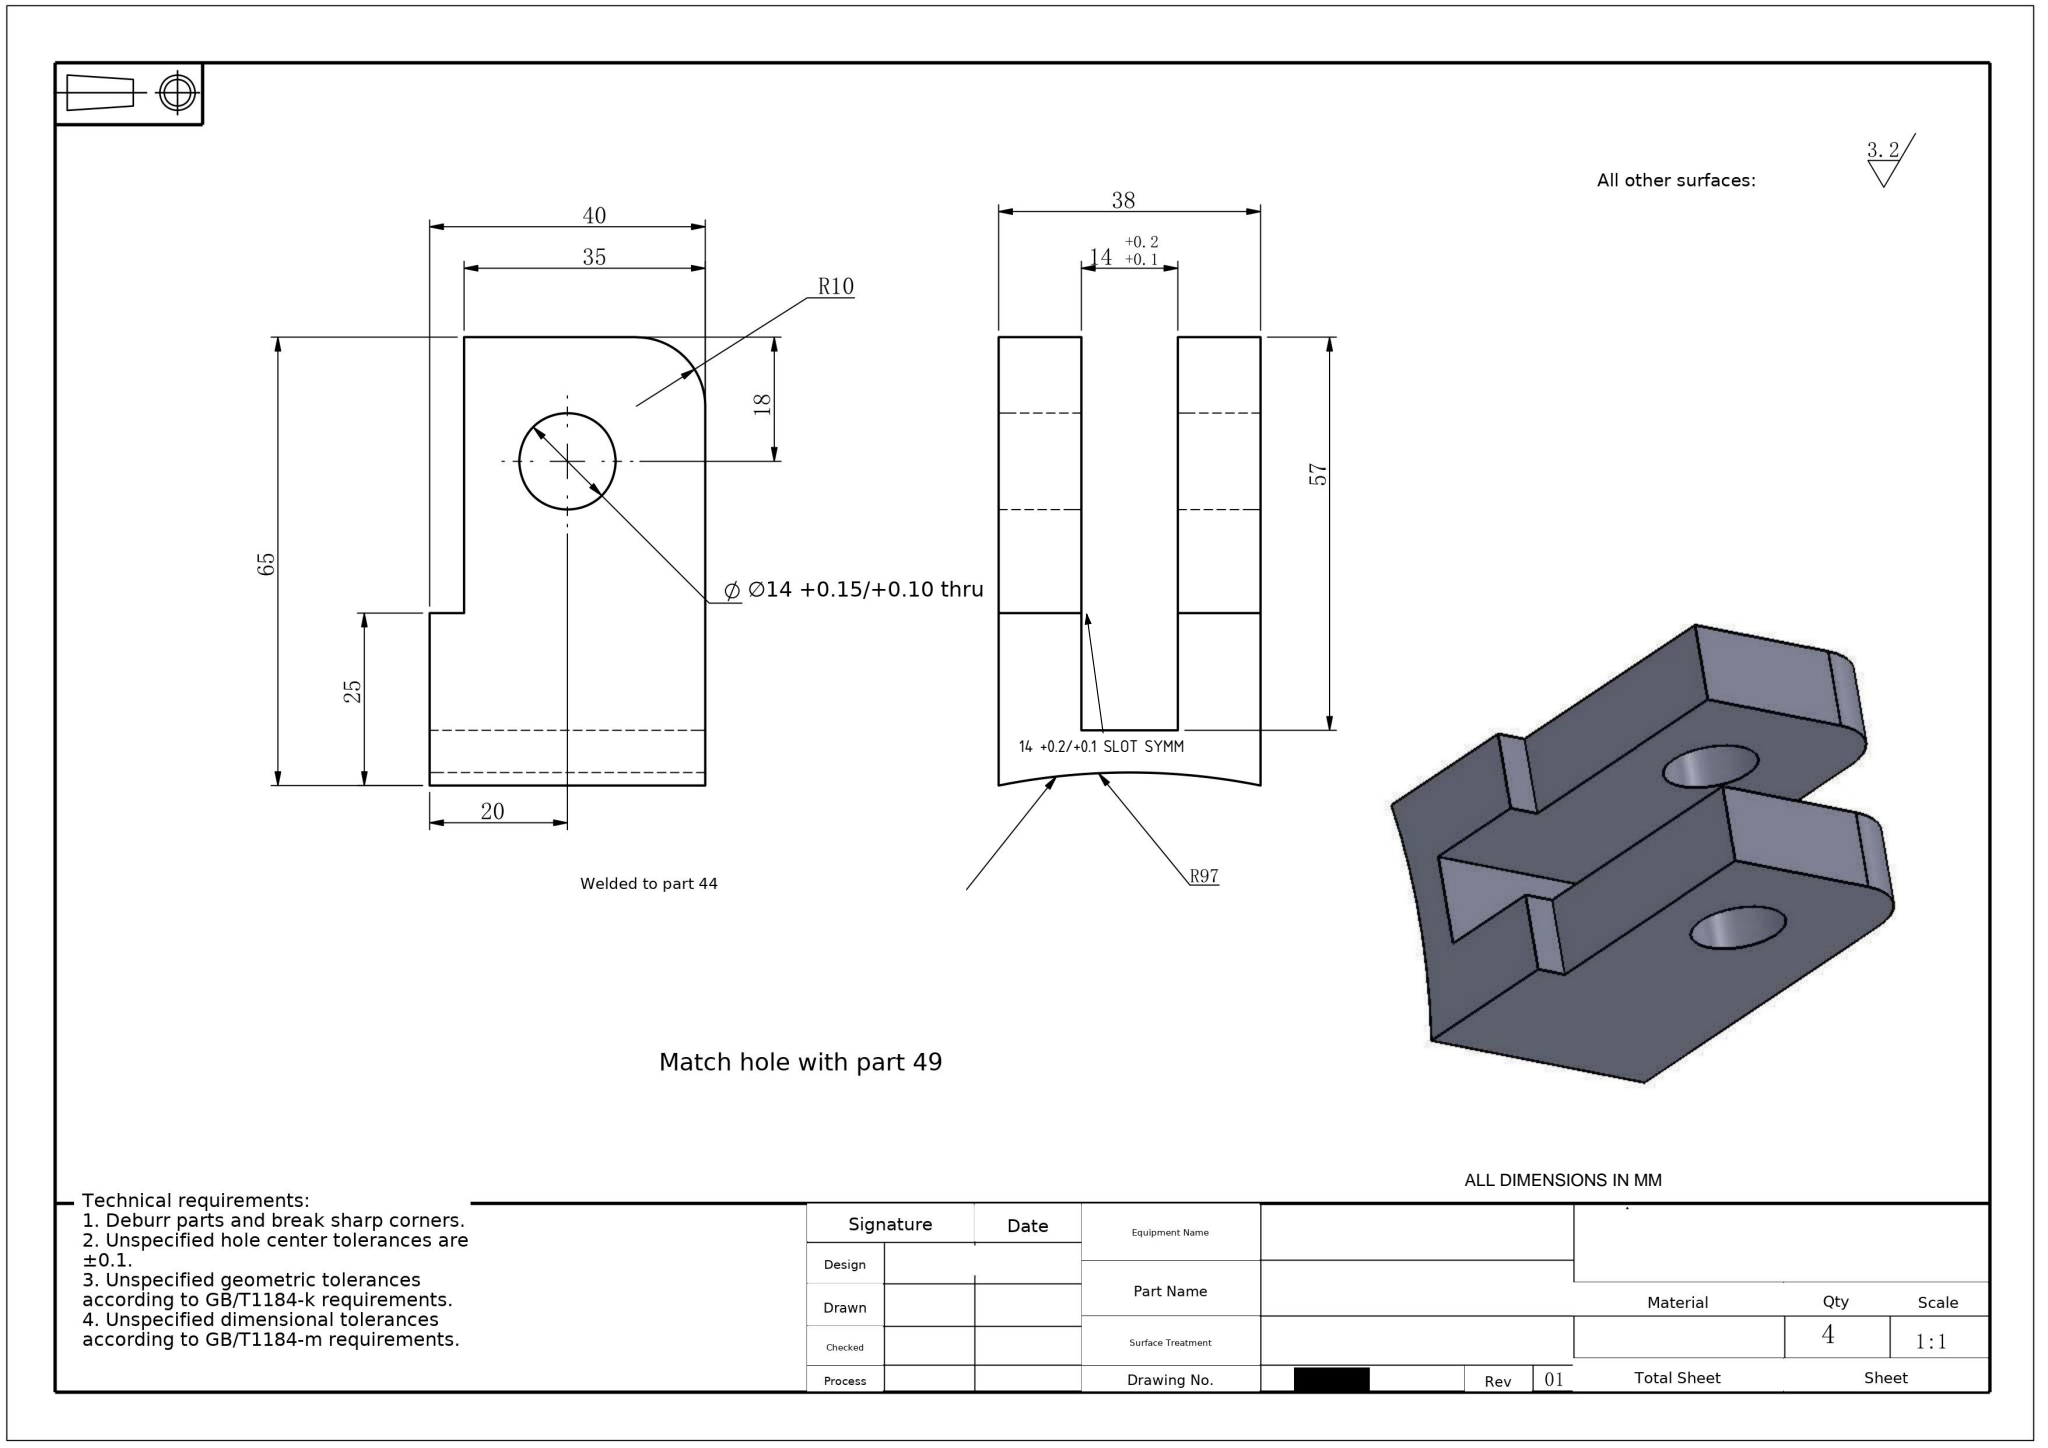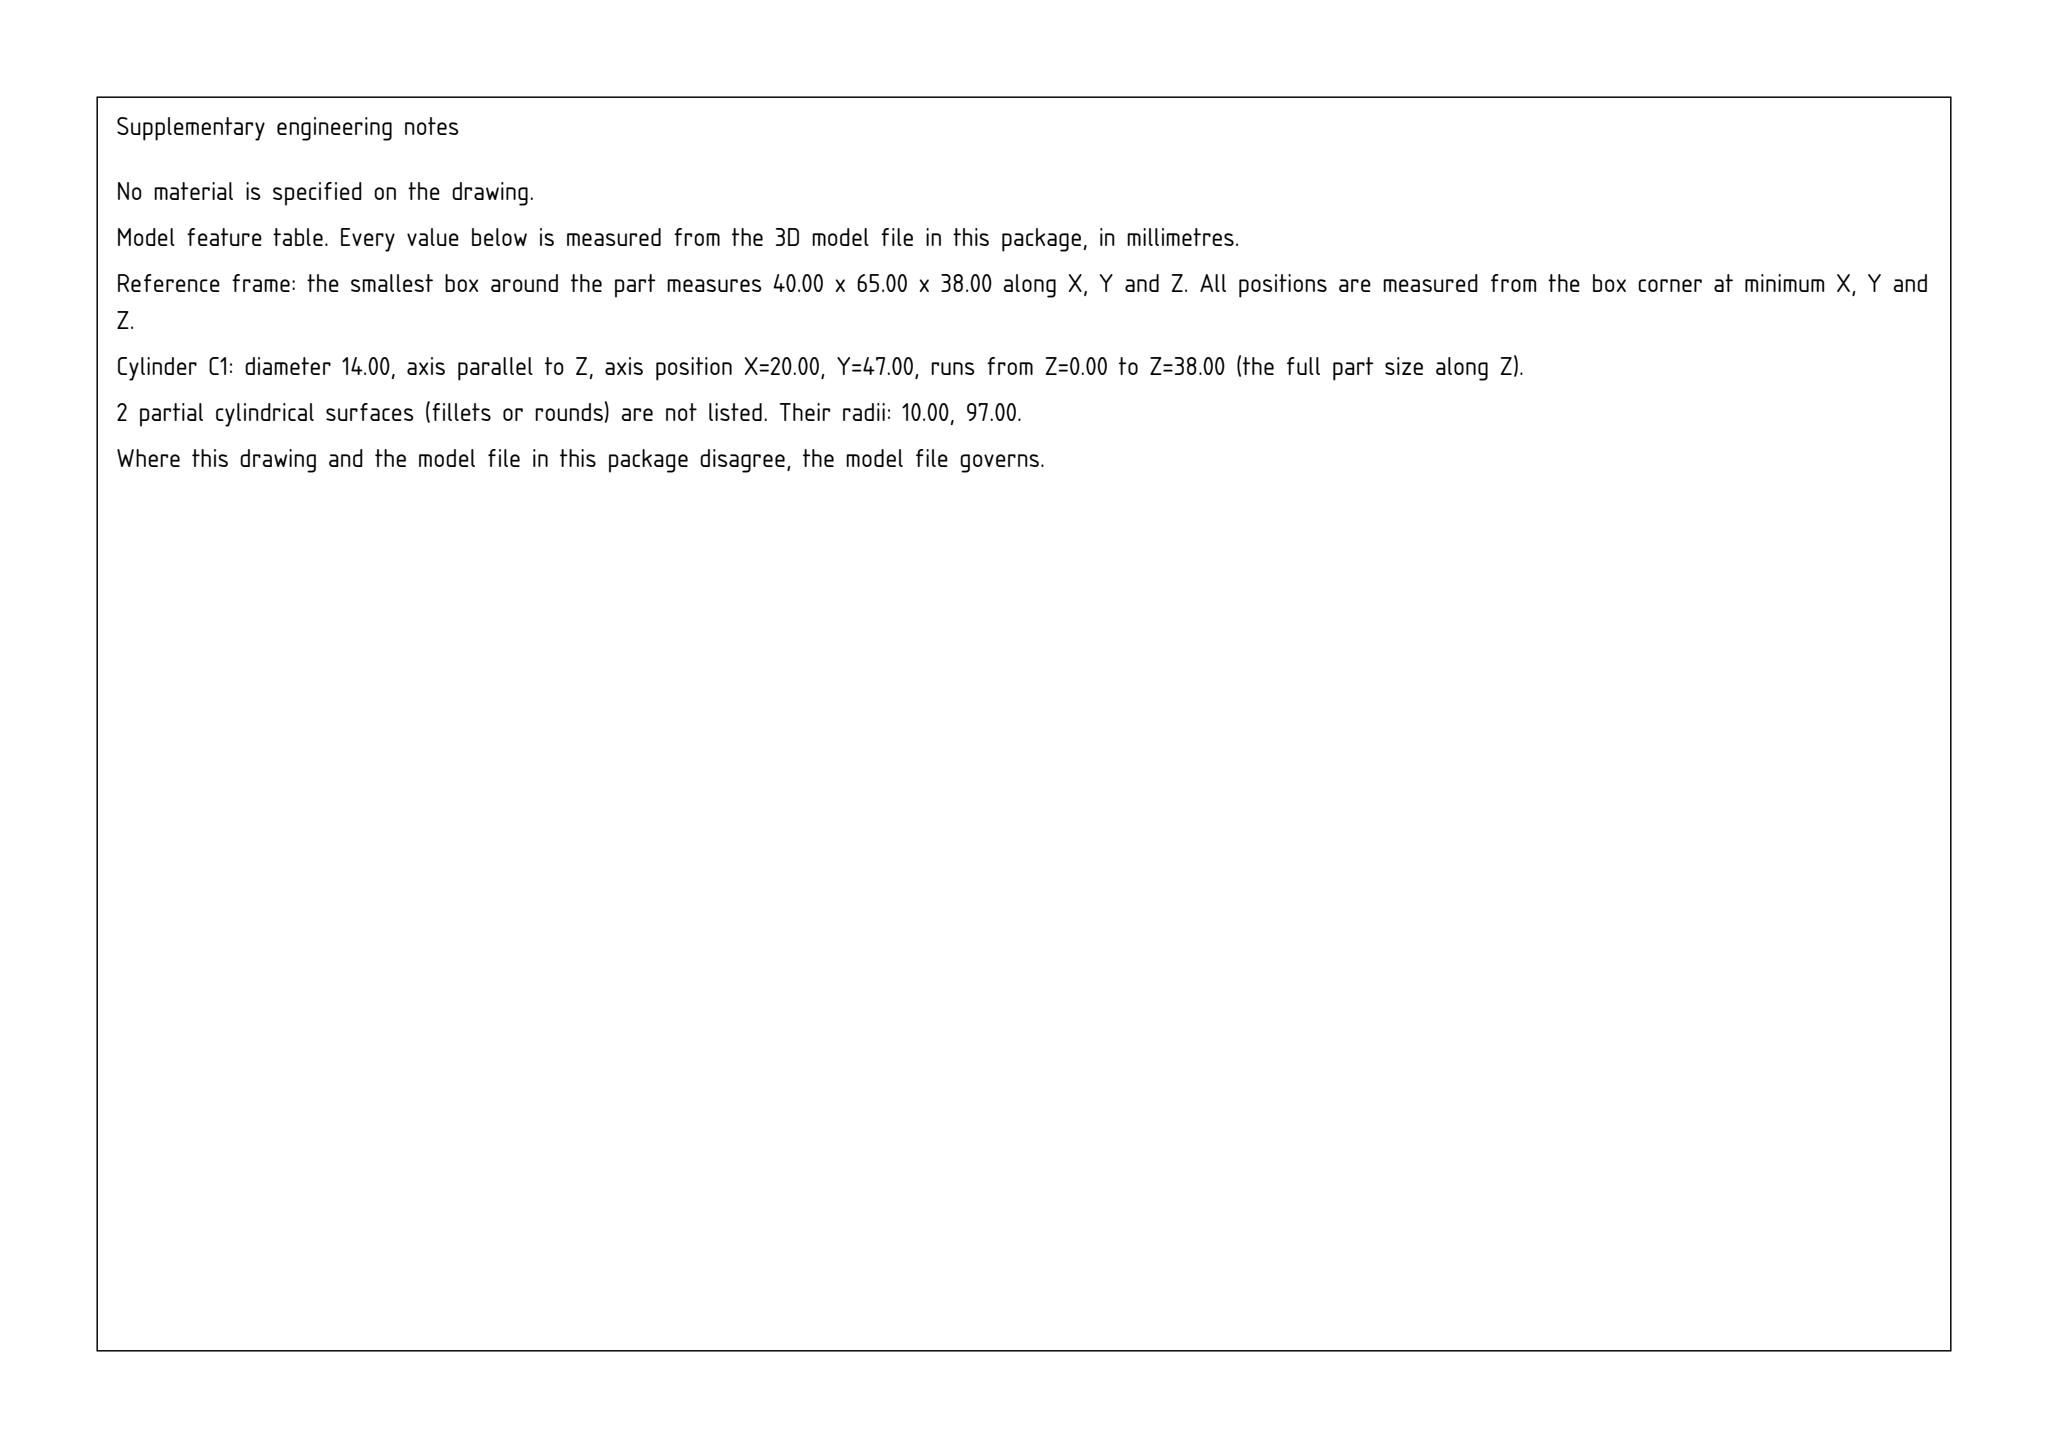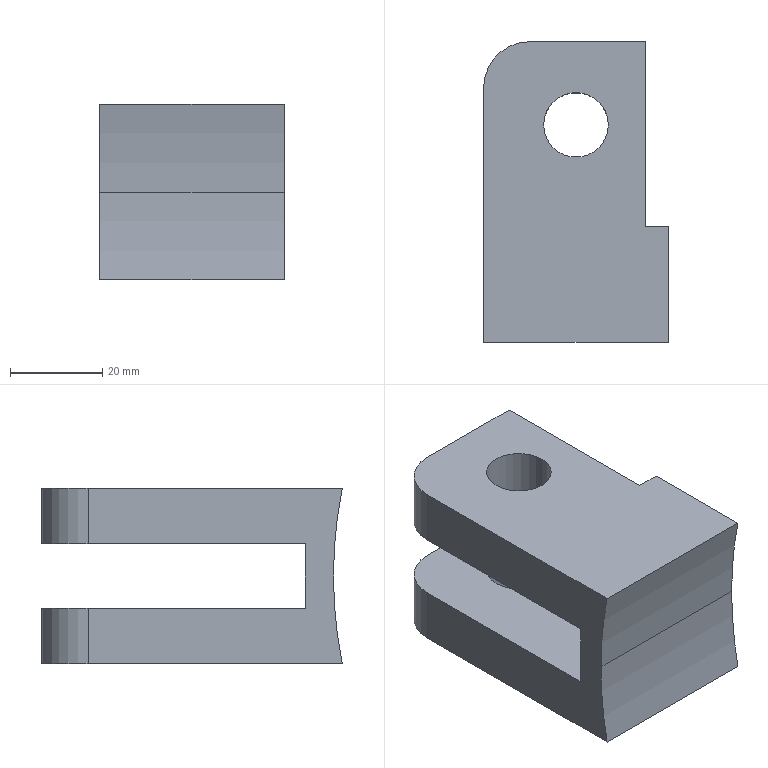Part | SolidWorks | mm | 1 solid | 21 faces | box 40 x 65 x 38 mm | volume 55963 mm3 | plane 13 | cylinder 8 | commonest cylinder face diameters 14 x4 194 x2 20 x2
Drawing notes:
14 +0.2/+0.1 SLOT SYMM ABOUT CL OF 38 THK: 12 FROM EA FACE | from the solid: z-planes at 12.0 and 26.0 within 38.0 thickness; slot width 14, centered at z=19=38/2
build123d program:
from build123d import *

# Parameters (mm, degrees)
BOSS_EXTRUDE1_DEPTH = 38
SKETCH2_R           = 7
CUT_EXTRUDE1_DEPTH  = 86.424
SKETCH3_W           = 14
SKETCH3_H           = 57
CUT_EXTRUDE2_DEPTH  = 67.334
SKETCH4_R           = 97
CUT_EXTRUDE3_DEPTH  = 67.334
FILLET1_R           = 10


with BuildPart() as part:
    # Sketch1 → Boss-Extrude1 (new body)
    with BuildSketch(Plane.XY):
        Polygon((-67.06, 28.173), (-32.06, 28.173), (-32.06, -11.827), (-27.06, -11.827), (-27.06, -36.827), (-67.06, -36.827), align=None)
    extrude(amount=BOSS_EXTRUDE1_DEPTH)

    # Sketch2 → Cut-Extrude1 (cut, through all)
    with BuildSketch(Plane.XY.offset(38)):
        with Locations((-47.06, 10.173)):
            Circle(SKETCH2_R)
    extrude(amount=-CUT_EXTRUDE1_DEPTH, mode=Mode.SUBTRACT)

    # Sketch3 → Cut-Extrude2 (cut, through all)
    with BuildSketch(Plane.ZY.offset(67.06)):
        with Locations((19, -0.3267)):
            Rectangle(SKETCH3_W, SKETCH3_H)
    extrude(amount=-CUT_EXTRUDE2_DEPTH, mode=Mode.SUBTRACT)

    # Sketch4 → Cut-Extrude3 (cut, through all)
    with BuildSketch(Plane(origin=(-27.06, 0, 0), x_dir=(0, 0, -1), z_dir=(1, 0, 0))):
        with Locations((-19, -131.948)):
            Circle(SKETCH4_R)
    extrude(amount=-CUT_EXTRUDE3_DEPTH, mode=Mode.SUBTRACT)

    # Fillet1
    fillet1_edges = [part.edges().sort_by_distance(p)[0] for p in [
        (-67.06, 28.173, 32),
        (-67.06, 28.173, 6),
    ]]
    fillet(fillet1_edges, radius=FILLET1_R)


solid = part.part
STEP:
#1=CARTESIAN_POINT('',(-67.06,-34.948,19.));
#2=VERTEX_POINT('',#1);
#3=CARTESIAN_POINT('',(-67.06,-36.827,38.));
#4=VERTEX_POINT('',#3);
#5=CARTESIAN_POINT('',(-67.06,-131.948,19.));
#6=DIRECTION('',(1.,0.,0.));
#7=DIRECTION('',(-0.,1.,0.));
#8=AXIS2_PLACEMENT_3D('',#5,#6,#7);
#9=CIRCLE('',#8,97.);
#10=EDGE_CURVE('',#2,#4,#9,.T.);
#11=ORIENTED_EDGE('',*,*,#10,.F.);
#12=CARTESIAN_POINT('',(-27.06,-34.948,19.));
#13=VERTEX_POINT('',#12);
#14=CARTESIAN_POINT('',(-67.06,-34.948,19.));
#15=DIRECTION('',(1.,0.,0.));
#16=VECTOR('',#15,1000.);
#17=LINE('',#14,#16);
#18=EDGE_CURVE('',#2,#13,#17,.T.);
#19=ORIENTED_EDGE('',*,*,#18,.T.);
#20=CARTESIAN_POINT('',(-27.06,-36.827,38.));
#21=VERTEX_POINT('',#20);
#22=CARTESIAN_POINT('',(-27.06,-131.948,19.));
#23=DIRECTION('',(1.,0.,0.));
#24=DIRECTION('',(-0.,1.,0.));
#25=AXIS2_PLACEMENT_3D('',#22,#23,#24);
#26=CIRCLE('',#25,97.);
#27=EDGE_CURVE('',#13,#21,#26,.T.);
#28=ORIENTED_EDGE('',*,*,#27,.T.);
#29=CARTESIAN_POINT('',(-27.06,-36.827,38.));
#30=DIRECTION('',(1.,0.,0.));
#31=VECTOR('',#30,1000.);
#32=LINE('',#29,#31);
#33=EDGE_CURVE('',#4,#21,#32,.T.);
#34=ORIENTED_EDGE('',*,*,#33,.F.);
#35=EDGE_LOOP('',(#11,#19,#28,#34));
#36=FACE_OUTER_BOUND('',#35,.T.);
#37=CARTESIAN_POINT('',(-67.06,-131.948,19.));
#38=DIRECTION('',(1.,0.,0.));
#39=DIRECTION('',(-0.,1.,0.));
#40=AXIS2_PLACEMENT_3D('',#37,#38,#39);
#41=CYLINDRICAL_SURFACE('',#40,97.);
#42=ADVANCED_FACE('',(#36),#41,.F.);
#43=CARTESIAN_POINT('',(-40.06,10.173,26.));
#44=VERTEX_POINT('',#43);
#45=CARTESIAN_POINT('',(-54.06,10.173,26.));
#46=VERTEX_POINT('',#45);
#47=CARTESIAN_POINT('',(-47.06,10.173,26.));
#48=DIRECTION('',(0.,-0.,-1.));
#49=DIRECTION('',(0.,-1.,0.));
#50=AXIS2_PLACEMENT_3D('',#47,#48,#49);
#51=CIRCLE('',#50,7.);
#52=EDGE_CURVE('',#44,#46,#51,.T.);
#53=ORIENTED_EDGE('',*,*,#52,.T.);
#54=CARTESIAN_POINT('',(-54.06,10.173,38.));
#55=VERTEX_POINT('',#54);
#56=CARTESIAN_POINT('',(-54.06,10.173,0.));
#57=DIRECTION('',(0.,0.,1.));
#58=VECTOR('',#57,1000.);
#59=LINE('',#56,#58);
#60=EDGE_CURVE('',#46,#55,#59,.T.);
#61=ORIENTED_EDGE('',*,*,#60,.T.);
#62=CARTESIAN_POINT('',(-40.06,10.173,38.));
#63=VERTEX_POINT('',#62);
#64=CARTESIAN_POINT('',(-47.06,10.173,38.));
#65=DIRECTION('',(0.,0.,1.));
#66=DIRECTION('',(1.,0.,0.));
#67=AXIS2_PLACEMENT_3D('',#64,#65,#66);
#68=CIRCLE('',#67,7.);
#69=EDGE_CURVE('',#55,#63,#68,.T.);
#70=ORIENTED_EDGE('',*,*,#69,.T.);
#71=CARTESIAN_POINT('',(-40.06,10.173,0.));
#72=DIRECTION('',(0.,0.,1.));
#73=VECTOR('',#72,1000.);
#74=LINE('',#71,#73);
#75=EDGE_CURVE('',#44,#63,#74,.T.);
#76=ORIENTED_EDGE('',*,*,#75,.F.);
#77=EDGE_LOOP('',(#53,#61,#70,#76));
#78=FACE_OUTER_BOUND('',#77,.T.);
#79=CARTESIAN_POINT('',(-47.06,10.173,0.));
#80=DIRECTION('',(0.,0.,1.));
#81=DIRECTION('',(1.,0.,0.));
#82=AXIS2_PLACEMENT_3D('',#79,#80,#81);
#83=CYLINDRICAL_SURFACE('',#82,7.);
#84=ADVANCED_FACE('',(#78),#83,.F.);
#85=CARTESIAN_POINT('',(-54.06,10.173,0.));
#86=VERTEX_POINT('',#85);
#87=CARTESIAN_POINT('',(-40.06,10.173,0.));
#88=VERTEX_POINT('',#87);
#89=CARTESIAN_POINT('',(-47.06,10.173,0.));
#90=DIRECTION('',(0.,0.,1.));
#91=DIRECTION('',(1.,0.,0.));
#92=AXIS2_PLACEMENT_3D('',#89,#90,#91);
#93=CIRCLE('',#92,7.);
#94=EDGE_CURVE('',#86,#88,#93,.T.);
#95=ORIENTED_EDGE('',*,*,#94,.F.);
#96=CARTESIAN_POINT('',(-54.06,10.173,12.));
#97=VERTEX_POINT('',#96);
#98=CARTESIAN_POINT('',(-54.06,10.173,0.));
#99=DIRECTION('',(0.,0.,1.));
#100=VECTOR('',#99,1000.);
#101=LINE('',#98,#100);
#102=EDGE_CURVE('',#86,#97,#101,.T.);
#103=ORIENTED_EDGE('',*,*,#102,.T.);
#104=CARTESIAN_POINT('',(-40.06,10.173,12.));
#105=VERTEX_POINT('',#104);
#106=CARTESIAN_POINT('',(-47.06,10.173,12.));
#107=DIRECTION('',(-0.,0.,1.));
#108=DIRECTION('',(0.,1.,0.));
#109=AXIS2_PLACEMENT_3D('',#106,#107,#108);
#110=CIRCLE('',#109,7.);
#111=EDGE_CURVE('',#97,#105,#110,.T.);
#112=ORIENTED_EDGE('',*,*,#111,.T.);
#113=CARTESIAN_POINT('',(-40.06,10.173,0.));
#114=DIRECTION('',(0.,0.,1.));
#115=VECTOR('',#114,1000.);
#116=LINE('',#113,#115);
#117=EDGE_CURVE('',#88,#105,#116,.T.);
#118=ORIENTED_EDGE('',*,*,#117,.F.);
#119=EDGE_LOOP('',(#95,#103,#112,#118));
#120=FACE_OUTER_BOUND('',#119,.T.);
#121=CARTESIAN_POINT('',(-47.06,10.173,0.));
#122=DIRECTION('',(0.,0.,1.));
#123=DIRECTION('',(1.,0.,0.));
#124=AXIS2_PLACEMENT_3D('',#121,#122,#123);
#125=CYLINDRICAL_SURFACE('',#124,7.);
#126=ADVANCED_FACE('',(#120),#125,.F.);
#127=CARTESIAN_POINT('',(-32.06,-11.827,12.));
#128=VERTEX_POINT('',#127);
#129=CARTESIAN_POINT('',(-32.06,-11.827,0.));
#130=VERTEX_POINT('',#129);
#131=CARTESIAN_POINT('',(-32.06,-11.827,38.));
#132=DIRECTION('',(0.,0.,-1.));
#133=VECTOR('',#132,1000.);
#134=LINE('',#131,#133);
#135=EDGE_CURVE('',#128,#130,#134,.T.);
#136=ORIENTED_EDGE('',*,*,#135,.F.);
#137=CARTESIAN_POINT('',(-27.06,-11.827,12.));
#138=VERTEX_POINT('',#137);
#139=CARTESIAN_POINT('',(-32.06,-11.827,12.));
#140=DIRECTION('',(1.,0.,-0.));
#141=VECTOR('',#140,1000.);
#142=LINE('',#139,#141);
#143=EDGE_CURVE('',#128,#138,#142,.T.);
#144=ORIENTED_EDGE('',*,*,#143,.T.);
#145=CARTESIAN_POINT('',(-27.06,-11.827,0.));
#146=VERTEX_POINT('',#145);
#147=CARTESIAN_POINT('',(-27.06,-11.827,38.));
#148=DIRECTION('',(0.,0.,-1.));
#149=VECTOR('',#148,1000.);
#150=LINE('',#147,#149);
#151=EDGE_CURVE('',#138,#146,#150,.T.);
#152=ORIENTED_EDGE('',*,*,#151,.T.);
#153=CARTESIAN_POINT('',(-32.06,-11.827,0.));
#154=DIRECTION('',(-1.,-0.,0.));
#155=VECTOR('',#154,1000.);
#156=LINE('',#153,#155);
#157=EDGE_CURVE('',#146,#130,#156,.T.);
#158=ORIENTED_EDGE('',*,*,#157,.T.);
#159=EDGE_LOOP('',(#136,#144,#152,#158));
#160=FACE_OUTER_BOUND('',#159,.T.);
#161=CARTESIAN_POINT('',(-32.06,-11.827,38.));
#162=DIRECTION('',(0.,-1.,0.));
#163=DIRECTION('',(1.,0.,0.));
#164=AXIS2_PLACEMENT_3D('',#161,#162,#163);
#165=PLANE('',#164);
#166=ADVANCED_FACE('',(#160),#165,.F.);
#167=CARTESIAN_POINT('',(-32.06,28.173,12.));
#168=VERTEX_POINT('',#167);
#169=CARTESIAN_POINT('',(-32.06,28.173,0.));
#170=VERTEX_POINT('',#169);
#171=CARTESIAN_POINT('',(-32.06,28.173,38.));
#172=DIRECTION('',(0.,0.,-1.));
#173=VECTOR('',#172,1000.);
#174=LINE('',#171,#173);
#175=EDGE_CURVE('',#168,#170,#174,.T.);
#176=ORIENTED_EDGE('',*,*,#175,.F.);
#177=CARTESIAN_POINT('',(-32.06,28.173,12.));
#178=DIRECTION('',(0.,-1.,0.));
#179=VECTOR('',#178,1000.);
#180=LINE('',#177,#179);
#181=EDGE_CURVE('',#168,#128,#180,.T.);
#182=ORIENTED_EDGE('',*,*,#181,.T.);
#183=ORIENTED_EDGE('',*,*,#135,.T.);
#184=CARTESIAN_POINT('',(-32.06,28.173,0.));
#185=DIRECTION('',(-0.,1.,0.));
#186=VECTOR('',#185,1000.);
#187=LINE('',#184,#186);
#188=EDGE_CURVE('',#130,#170,#187,.T.);
#189=ORIENTED_EDGE('',*,*,#188,.T.);
#190=EDGE_LOOP('',(#176,#182,#183,#189));
#191=FACE_OUTER_BOUND('',#190,.T.);
#192=CARTESIAN_POINT('',(-32.06,28.173,38.));
#193=DIRECTION('',(-1.,-0.,0.));
#194=DIRECTION('',(0.,-1.,0.));
#195=AXIS2_PLACEMENT_3D('',#192,#193,#194);
#196=PLANE('',#195);
#197=ADVANCED_FACE('',(#191),#196,.F.);
#198=CARTESIAN_POINT('',(-57.06,28.173,0.));
#199=VERTEX_POINT('',#198);
#200=CARTESIAN_POINT('',(-67.06,28.173,0.));
#201=DIRECTION('',(-1.,0.,0.));
#202=VECTOR('',#201,1000.);
#203=LINE('',#200,#202);
#204=EDGE_CURVE('',#170,#199,#203,.T.);
#205=ORIENTED_EDGE('',*,*,#204,.T.);
#206=CARTESIAN_POINT('',(-57.06,28.173,12.));
#207=VERTEX_POINT('',#206);
#208=CARTESIAN_POINT('',(-57.06,28.173,38.));
#209=DIRECTION('',(0.,0.,1.));
#210=VECTOR('',#209,1000.);
#211=LINE('',#208,#210);
#212=EDGE_CURVE('',#199,#207,#211,.T.);
#213=ORIENTED_EDGE('',*,*,#212,.T.);
#214=CARTESIAN_POINT('',(-27.06,28.173,12.));
#215=DIRECTION('',(-1.,-0.,0.));
#216=VECTOR('',#215,1000.);
#217=LINE('',#214,#216);
#218=EDGE_CURVE('',#168,#207,#217,.T.);
#219=ORIENTED_EDGE('',*,*,#218,.F.);
#220=ORIENTED_EDGE('',*,*,#175,.T.);
#221=EDGE_LOOP('',(#205,#213,#219,#220));
#222=FACE_OUTER_BOUND('',#221,.T.);
#223=CARTESIAN_POINT('',(-67.06,28.173,38.));
#224=DIRECTION('',(0.,-1.,0.));
#225=DIRECTION('',(0.,0.,-1.));
#226=AXIS2_PLACEMENT_3D('',#223,#224,#225);
#227=PLANE('',#226);
#228=ADVANCED_FACE('',(#222),#227,.F.);
#229=ORIENTED_EDGE('',*,*,#102,.F.);
#230=CARTESIAN_POINT('',(-47.06,10.173,0.));
#231=DIRECTION('',(0.,0.,1.));
#232=DIRECTION('',(1.,0.,0.));
#233=AXIS2_PLACEMENT_3D('',#230,#231,#232);
#234=CIRCLE('',#233,7.);
#235=EDGE_CURVE('',#88,#86,#234,.T.);
#236=ORIENTED_EDGE('',*,*,#235,.F.);
#237=ORIENTED_EDGE('',*,*,#117,.T.);
#238=CARTESIAN_POINT('',(-47.06,10.173,12.));
#239=DIRECTION('',(-0.,0.,1.));
#240=DIRECTION('',(0.,1.,0.));
#241=AXIS2_PLACEMENT_3D('',#238,#239,#240);
#242=CIRCLE('',#241,7.);
#243=EDGE_CURVE('',#105,#97,#242,.T.);
#244=ORIENTED_EDGE('',*,*,#243,.T.);
#245=EDGE_LOOP('',(#229,#236,#237,#244));
#246=FACE_OUTER_BOUND('',#245,.T.);
#247=CARTESIAN_POINT('',(-47.06,10.173,0.));
#248=DIRECTION('',(0.,0.,1.));
#249=DIRECTION('',(1.,0.,0.));
#250=AXIS2_PLACEMENT_3D('',#247,#248,#249);
#251=CYLINDRICAL_SURFACE('',#250,7.);
#252=ADVANCED_FACE('',(#246),#251,.F.);
#253=CARTESIAN_POINT('',(-67.06,18.173,12.));
#254=VERTEX_POINT('',#253);
#255=CARTESIAN_POINT('',(-67.06,-28.827,12.));
#256=VERTEX_POINT('',#255);
#257=CARTESIAN_POINT('',(-67.06,28.173,12.));
#258=DIRECTION('',(0.,-1.,0.));
#259=VECTOR('',#258,1000.);
#260=LINE('',#257,#259);
#261=EDGE_CURVE('',#254,#256,#260,.T.);
#262=ORIENTED_EDGE('',*,*,#261,.F.);
#263=CARTESIAN_POINT('',(-67.06,18.173,0.));
#264=VERTEX_POINT('',#263);
#265=CARTESIAN_POINT('',(-67.06,18.173,38.));
#266=DIRECTION('',(0.,0.,-1.));
#267=VECTOR('',#266,1000.);
#268=LINE('',#265,#267);
#269=EDGE_CURVE('',#254,#264,#268,.T.);
#270=ORIENTED_EDGE('',*,*,#269,.T.);
#271=CARTESIAN_POINT('',(-67.06,-36.827,0.));
#272=VERTEX_POINT('',#271);
#273=CARTESIAN_POINT('',(-67.06,28.173,0.));
#274=DIRECTION('',(0.,-1.,0.));
#275=VECTOR('',#274,1000.);
#276=LINE('',#273,#275);
#277=EDGE_CURVE('',#264,#272,#276,.T.);
#278=ORIENTED_EDGE('',*,*,#277,.T.);
#279=CARTESIAN_POINT('',(-67.06,-131.948,19.));
#280=DIRECTION('',(1.,0.,0.));
#281=DIRECTION('',(-0.,1.,0.));
#282=AXIS2_PLACEMENT_3D('',#279,#280,#281);
#283=CIRCLE('',#282,97.);
#284=EDGE_CURVE('',#272,#2,#283,.T.);
#285=ORIENTED_EDGE('',*,*,#284,.T.);
#286=ORIENTED_EDGE('',*,*,#10,.T.);
#287=CARTESIAN_POINT('',(-67.06,18.173,38.));
#288=VERTEX_POINT('',#287);
#289=CARTESIAN_POINT('',(-67.06,28.173,38.));
#290=DIRECTION('',(0.,-1.,0.));
#291=VECTOR('',#290,1000.);
#292=LINE('',#289,#291);
#293=EDGE_CURVE('',#288,#4,#292,.T.);
#294=ORIENTED_EDGE('',*,*,#293,.F.);
#295=CARTESIAN_POINT('',(-67.06,18.173,26.));
#296=VERTEX_POINT('',#295);
#297=CARTESIAN_POINT('',(-67.06,18.173,38.));
#298=DIRECTION('',(0.,0.,-1.));
#299=VECTOR('',#298,1000.);
#300=LINE('',#297,#299);
#301=EDGE_CURVE('',#288,#296,#300,.T.);
#302=ORIENTED_EDGE('',*,*,#301,.T.);
#303=CARTESIAN_POINT('',(-67.06,-28.827,26.));
#304=VERTEX_POINT('',#303);
#305=CARTESIAN_POINT('',(-67.06,28.173,26.));
#306=DIRECTION('',(0.,1.,-0.));
#307=VECTOR('',#306,1000.);
#308=LINE('',#305,#307);
#309=EDGE_CURVE('',#304,#296,#308,.T.);
#310=ORIENTED_EDGE('',*,*,#309,.F.);
#311=CARTESIAN_POINT('',(-67.06,-28.827,12.));
#312=DIRECTION('',(0.,0.,1.));
#313=VECTOR('',#312,1000.);
#314=LINE('',#311,#313);
#315=EDGE_CURVE('',#256,#304,#314,.T.);
#316=ORIENTED_EDGE('',*,*,#315,.F.);
#317=EDGE_LOOP('',(#262,#270,#278,#285,#286,#294,#302,#310,#316));
#318=FACE_OUTER_BOUND('',#317,.T.);
#319=CARTESIAN_POINT('',(-67.06,28.173,38.));
#320=DIRECTION('',(1.,0.,0.));
#321=DIRECTION('',(-0.,1.,0.));
#322=AXIS2_PLACEMENT_3D('',#319,#320,#321);
#323=PLANE('',#322);
#324=ADVANCED_FACE('',(#318),#323,.F.);
#325=CARTESIAN_POINT('',(-27.06,-11.827,38.));
#326=VERTEX_POINT('',#325);
#327=CARTESIAN_POINT('',(-27.06,-11.827,38.));
#328=DIRECTION('',(-0.,1.,0.));
#329=VECTOR('',#328,1000.);
#330=LINE('',#327,#329);
#331=EDGE_CURVE('',#21,#326,#330,.T.);
#332=ORIENTED_EDGE('',*,*,#331,.F.);
#333=ORIENTED_EDGE('',*,*,#27,.F.);
#334=CARTESIAN_POINT('',(-27.06,-36.827,0.));
#335=VERTEX_POINT('',#334);
#336=CARTESIAN_POINT('',(-27.06,-131.948,19.));
#337=DIRECTION('',(1.,0.,0.));
#338=DIRECTION('',(-0.,1.,0.));
#339=AXIS2_PLACEMENT_3D('',#336,#337,#338);
#340=CIRCLE('',#339,97.);
#341=EDGE_CURVE('',#335,#13,#340,.T.);
#342=ORIENTED_EDGE('',*,*,#341,.F.);
#343=CARTESIAN_POINT('',(-27.06,-11.827,0.));
#344=DIRECTION('',(-0.,1.,0.));
#345=VECTOR('',#344,1000.);
#346=LINE('',#343,#345);
#347=EDGE_CURVE('',#335,#146,#346,.T.);
#348=ORIENTED_EDGE('',*,*,#347,.T.);
#349=ORIENTED_EDGE('',*,*,#151,.F.);
#350=CARTESIAN_POINT('',(-27.06,-28.827,12.));
#351=VERTEX_POINT('',#350);
#352=CARTESIAN_POINT('',(-27.06,28.173,12.));
#353=DIRECTION('',(0.,-1.,0.));
#354=VECTOR('',#353,1000.);
#355=LINE('',#352,#354);
#356=EDGE_CURVE('',#138,#351,#355,.T.);
#357=ORIENTED_EDGE('',*,*,#356,.T.);
#358=CARTESIAN_POINT('',(-27.06,-28.827,26.));
#359=VERTEX_POINT('',#358);
#360=CARTESIAN_POINT('',(-27.06,-28.827,12.));
#361=DIRECTION('',(0.,0.,1.));
#362=VECTOR('',#361,1000.);
#363=LINE('',#360,#362);
#364=EDGE_CURVE('',#351,#359,#363,.T.);
#365=ORIENTED_EDGE('',*,*,#364,.T.);
#366=CARTESIAN_POINT('',(-27.06,-11.827,26.));
#367=VERTEX_POINT('',#366);
#368=CARTESIAN_POINT('',(-27.06,28.173,26.));
#369=DIRECTION('',(0.,1.,-0.));
#370=VECTOR('',#369,1000.);
#371=LINE('',#368,#370);
#372=EDGE_CURVE('',#359,#367,#371,.T.);
#373=ORIENTED_EDGE('',*,*,#372,.T.);
#374=CARTESIAN_POINT('',(-27.06,-11.827,38.));
#375=DIRECTION('',(0.,0.,-1.));
#376=VECTOR('',#375,1000.);
#377=LINE('',#374,#376);
#378=EDGE_CURVE('',#326,#367,#377,.T.);
#379=ORIENTED_EDGE('',*,*,#378,.F.);
#380=EDGE_LOOP('',(#332,#333,#342,#348,#349,#357,#365,#373,#379));
#381=FACE_OUTER_BOUND('',#380,.T.);
#382=CARTESIAN_POINT('',(-27.06,-11.827,38.));
#383=DIRECTION('',(-1.,-0.,0.));
#384=DIRECTION('',(0.,-1.,0.));
#385=AXIS2_PLACEMENT_3D('',#382,#383,#384);
#386=PLANE('',#385);
#387=ADVANCED_FACE('',(#381),#386,.F.);
#388=ORIENTED_EDGE('',*,*,#378,.T.);
#389=CARTESIAN_POINT('',(-32.06,-11.827,26.));
#390=VERTEX_POINT('',#389);
#391=CARTESIAN_POINT('',(-32.06,-11.827,26.));
#392=DIRECTION('',(-1.,-0.,0.));
#393=VECTOR('',#392,1000.);
#394=LINE('',#391,#393);
#395=EDGE_CURVE('',#367,#390,#394,.T.);
#396=ORIENTED_EDGE('',*,*,#395,.T.);
#397=CARTESIAN_POINT('',(-32.06,-11.827,38.));
#398=VERTEX_POINT('',#397);
#399=CARTESIAN_POINT('',(-32.06,-11.827,38.));
#400=DIRECTION('',(0.,0.,-1.));
#401=VECTOR('',#400,1000.);
#402=LINE('',#399,#401);
#403=EDGE_CURVE('',#398,#390,#402,.T.);
#404=ORIENTED_EDGE('',*,*,#403,.F.);
#405=CARTESIAN_POINT('',(-32.06,-11.827,38.));
#406=DIRECTION('',(-1.,-0.,0.));
#407=VECTOR('',#406,1000.);
#408=LINE('',#405,#407);
#409=EDGE_CURVE('',#326,#398,#408,.T.);
#410=ORIENTED_EDGE('',*,*,#409,.F.);
#411=EDGE_LOOP('',(#388,#396,#404,#410));
#412=FACE_OUTER_BOUND('',#411,.T.);
#413=CARTESIAN_POINT('',(-32.06,-11.827,38.));
#414=DIRECTION('',(0.,-1.,0.));
#415=DIRECTION('',(1.,0.,0.));
#416=AXIS2_PLACEMENT_3D('',#413,#414,#415);
#417=PLANE('',#416);
#418=ADVANCED_FACE('',(#412),#417,.F.);
#419=ORIENTED_EDGE('',*,*,#403,.T.);
#420=CARTESIAN_POINT('',(-32.06,28.173,26.));
#421=VERTEX_POINT('',#420);
#422=CARTESIAN_POINT('',(-32.06,28.173,26.));
#423=DIRECTION('',(-0.,1.,-0.));
#424=VECTOR('',#423,1000.);
#425=LINE('',#422,#424);
#426=EDGE_CURVE('',#390,#421,#425,.T.);
#427=ORIENTED_EDGE('',*,*,#426,.T.);
#428=CARTESIAN_POINT('',(-32.06,28.173,38.));
#429=VERTEX_POINT('',#428);
#430=CARTESIAN_POINT('',(-32.06,28.173,38.));
#431=DIRECTION('',(0.,0.,-1.));
#432=VECTOR('',#431,1000.);
#433=LINE('',#430,#432);
#434=EDGE_CURVE('',#429,#421,#433,.T.);
#435=ORIENTED_EDGE('',*,*,#434,.F.);
#436=CARTESIAN_POINT('',(-32.06,28.173,38.));
#437=DIRECTION('',(-0.,1.,0.));
#438=VECTOR('',#437,1000.);
#439=LINE('',#436,#438);
#440=EDGE_CURVE('',#398,#429,#439,.T.);
#441=ORIENTED_EDGE('',*,*,#440,.F.);
#442=EDGE_LOOP('',(#419,#427,#435,#441));
#443=FACE_OUTER_BOUND('',#442,.T.);
#444=CARTESIAN_POINT('',(-32.06,28.173,38.));
#445=DIRECTION('',(-1.,-0.,0.));
#446=DIRECTION('',(0.,-1.,0.));
#447=AXIS2_PLACEMENT_3D('',#444,#445,#446);
#448=PLANE('',#447);
#449=ADVANCED_FACE('',(#443),#448,.F.);
#450=CARTESIAN_POINT('',(-57.06,28.173,26.));
#451=VERTEX_POINT('',#450);
#452=CARTESIAN_POINT('',(-27.06,28.173,26.));
#453=DIRECTION('',(-1.,-0.,0.));
#454=VECTOR('',#453,1000.);
#455=LINE('',#452,#454);
#456=EDGE_CURVE('',#421,#451,#455,.T.);
#457=ORIENTED_EDGE('',*,*,#456,.T.);
#458=CARTESIAN_POINT('',(-57.06,28.173,38.));
#459=VERTEX_POINT('',#458);
#460=CARTESIAN_POINT('',(-57.06,28.173,38.));
#461=DIRECTION('',(0.,0.,1.));
#462=VECTOR('',#461,1000.);
#463=LINE('',#460,#462);
#464=EDGE_CURVE('',#451,#459,#463,.T.);
#465=ORIENTED_EDGE('',*,*,#464,.T.);
#466=CARTESIAN_POINT('',(-67.06,28.173,38.));
#467=DIRECTION('',(-1.,0.,0.));
#468=VECTOR('',#467,1000.);
#469=LINE('',#466,#468);
#470=EDGE_CURVE('',#429,#459,#469,.T.);
#471=ORIENTED_EDGE('',*,*,#470,.F.);
#472=ORIENTED_EDGE('',*,*,#434,.T.);
#473=EDGE_LOOP('',(#457,#465,#471,#472));
#474=FACE_OUTER_BOUND('',#473,.T.);
#475=CARTESIAN_POINT('',(-67.06,28.173,38.));
#476=DIRECTION('',(0.,-1.,0.));
#477=DIRECTION('',(0.,0.,-1.));
#478=AXIS2_PLACEMENT_3D('',#475,#476,#477);
#479=PLANE('',#478);
#480=ADVANCED_FACE('',(#474),#479,.F.);
#481=CARTESIAN_POINT('',(-47.06,10.173,38.));
#482=DIRECTION('',(0.,0.,1.));
#483=DIRECTION('',(1.,0.,0.));
#484=AXIS2_PLACEMENT_3D('',#481,#482,#483);
#485=CIRCLE('',#484,7.);
#486=EDGE_CURVE('',#63,#55,#485,.T.);
#487=ORIENTED_EDGE('',*,*,#486,.F.);
#488=ORIENTED_EDGE('',*,*,#69,.F.);
#489=EDGE_LOOP('',(#487,#488));
#490=FACE_BOUND('',#489,.T.);
#491=ORIENTED_EDGE('',*,*,#470,.T.);
#492=CARTESIAN_POINT('',(-57.06,18.173,38.));
#493=DIRECTION('',(0.,0.,1.));
#494=DIRECTION('',(-1.,0.,0.));
#495=AXIS2_PLACEMENT_3D('',#492,#493,#494);
#496=CIRCLE('',#495,10.);
#497=EDGE_CURVE('',#459,#288,#496,.T.);
#498=ORIENTED_EDGE('',*,*,#497,.T.);
#499=ORIENTED_EDGE('',*,*,#293,.T.);
#500=ORIENTED_EDGE('',*,*,#33,.T.);
#501=ORIENTED_EDGE('',*,*,#331,.T.);
#502=ORIENTED_EDGE('',*,*,#409,.T.);
#503=ORIENTED_EDGE('',*,*,#440,.T.);
#504=EDGE_LOOP('',(#491,#498,#499,#500,#501,#502,#503));
#505=FACE_OUTER_BOUND('',#504,.T.);
#506=CARTESIAN_POINT('',(-67.06,-36.827,38.));
#507=DIRECTION('',(0.,0.,-1.));
#508=DIRECTION('',(-1.,0.,0.));
#509=AXIS2_PLACEMENT_3D('',#506,#507,#508);
#510=PLANE('',#509);
#511=ADVANCED_FACE('',(#490,#505),#510,.F.);
#512=ORIENTED_EDGE('',*,*,#235,.T.);
#513=ORIENTED_EDGE('',*,*,#94,.T.);
#514=EDGE_LOOP('',(#512,#513));
#515=FACE_BOUND('',#514,.T.);
#516=ORIENTED_EDGE('',*,*,#277,.F.);
#517=CARTESIAN_POINT('',(-57.06,18.173,0.));
#518=DIRECTION('',(0.,0.,-1.));
#519=DIRECTION('',(-1.,0.,0.));
#520=AXIS2_PLACEMENT_3D('',#517,#518,#519);
#521=CIRCLE('',#520,10.);
#522=EDGE_CURVE('',#264,#199,#521,.T.);
#523=ORIENTED_EDGE('',*,*,#522,.T.);
#524=ORIENTED_EDGE('',*,*,#204,.F.);
#525=ORIENTED_EDGE('',*,*,#188,.F.);
#526=ORIENTED_EDGE('',*,*,#157,.F.);
#527=ORIENTED_EDGE('',*,*,#347,.F.);
#528=CARTESIAN_POINT('',(-27.06,-36.827,0.));
#529=DIRECTION('',(1.,0.,0.));
#530=VECTOR('',#529,1000.);
#531=LINE('',#528,#530);
#532=EDGE_CURVE('',#272,#335,#531,.T.);
#533=ORIENTED_EDGE('',*,*,#532,.F.);
#534=EDGE_LOOP('',(#516,#523,#524,#525,#526,#527,#533));
#535=FACE_OUTER_BOUND('',#534,.T.);
#536=CARTESIAN_POINT('',(-67.06,-36.827,0.));
#537=DIRECTION('',(0.,0.,-1.));
#538=DIRECTION('',(-1.,0.,0.));
#539=AXIS2_PLACEMENT_3D('',#536,#537,#538);
#540=PLANE('',#539);
#541=ADVANCED_FACE('',(#515,#535),#540,.T.);
#542=ORIENTED_EDGE('',*,*,#60,.F.);
#543=CARTESIAN_POINT('',(-47.06,10.173,26.));
#544=DIRECTION('',(0.,-0.,-1.));
#545=DIRECTION('',(0.,-1.,0.));
#546=AXIS2_PLACEMENT_3D('',#543,#544,#545);
#547=CIRCLE('',#546,7.);
#548=EDGE_CURVE('',#46,#44,#547,.T.);
#549=ORIENTED_EDGE('',*,*,#548,.T.);
#550=ORIENTED_EDGE('',*,*,#75,.T.);
#551=ORIENTED_EDGE('',*,*,#486,.T.);
#552=EDGE_LOOP('',(#542,#549,#550,#551));
#553=FACE_OUTER_BOUND('',#552,.T.);
#554=CARTESIAN_POINT('',(-47.06,10.173,0.));
#555=DIRECTION('',(0.,0.,1.));
#556=DIRECTION('',(1.,0.,0.));
#557=AXIS2_PLACEMENT_3D('',#554,#555,#556);
#558=CYLINDRICAL_SURFACE('',#557,7.);
#559=ADVANCED_FACE('',(#553),#558,.F.);
#560=ORIENTED_EDGE('',*,*,#243,.F.);
#561=ORIENTED_EDGE('',*,*,#111,.F.);
#562=EDGE_LOOP('',(#560,#561));
#563=FACE_BOUND('',#562,.T.);
#564=ORIENTED_EDGE('',*,*,#218,.T.);
#565=CARTESIAN_POINT('',(-57.06,18.173,12.));
#566=DIRECTION('',(-0.,0.,1.));
#567=DIRECTION('',(0.,1.,-0.));
#568=AXIS2_PLACEMENT_3D('',#565,#566,#567);
#569=CIRCLE('',#568,10.);
#570=EDGE_CURVE('',#207,#254,#569,.T.);
#571=ORIENTED_EDGE('',*,*,#570,.T.);
#572=ORIENTED_EDGE('',*,*,#261,.T.);
#573=CARTESIAN_POINT('',(-27.06,-28.827,12.));
#574=DIRECTION('',(-1.,-0.,0.));
#575=VECTOR('',#574,1000.);
#576=LINE('',#573,#575);
#577=EDGE_CURVE('',#351,#256,#576,.T.);
#578=ORIENTED_EDGE('',*,*,#577,.F.);
#579=ORIENTED_EDGE('',*,*,#356,.F.);
#580=ORIENTED_EDGE('',*,*,#143,.F.);
#581=ORIENTED_EDGE('',*,*,#181,.F.);
#582=EDGE_LOOP('',(#564,#571,#572,#578,#579,#580,#581));
#583=FACE_OUTER_BOUND('',#582,.T.);
#584=CARTESIAN_POINT('',(-27.06,28.173,12.));
#585=DIRECTION('',(0.,-0.,-1.));
#586=DIRECTION('',(0.,1.,-0.));
#587=AXIS2_PLACEMENT_3D('',#584,#585,#586);
#588=PLANE('',#587);
#589=ADVANCED_FACE('',(#563,#583),#588,.F.);
#590=ORIENTED_EDGE('',*,*,#52,.F.);
#591=ORIENTED_EDGE('',*,*,#548,.F.);
#592=EDGE_LOOP('',(#590,#591));
#593=FACE_BOUND('',#592,.T.);
#594=ORIENTED_EDGE('',*,*,#309,.T.);
#595=CARTESIAN_POINT('',(-57.06,18.173,26.));
#596=DIRECTION('',(0.,-0.,-1.));
#597=DIRECTION('',(0.,-1.,0.));
#598=AXIS2_PLACEMENT_3D('',#595,#596,#597);
#599=CIRCLE('',#598,10.);
#600=EDGE_CURVE('',#296,#451,#599,.T.);
#601=ORIENTED_EDGE('',*,*,#600,.T.);
#602=ORIENTED_EDGE('',*,*,#456,.F.);
#603=ORIENTED_EDGE('',*,*,#426,.F.);
#604=ORIENTED_EDGE('',*,*,#395,.F.);
#605=ORIENTED_EDGE('',*,*,#372,.F.);
#606=CARTESIAN_POINT('',(-27.06,-28.827,26.));
#607=DIRECTION('',(-1.,-0.,0.));
#608=VECTOR('',#607,1000.);
#609=LINE('',#606,#608);
#610=EDGE_CURVE('',#359,#304,#609,.T.);
#611=ORIENTED_EDGE('',*,*,#610,.T.);
#612=EDGE_LOOP('',(#594,#601,#602,#603,#604,#605,#611));
#613=FACE_OUTER_BOUND('',#612,.T.);
#614=CARTESIAN_POINT('',(-27.06,28.173,26.));
#615=DIRECTION('',(-0.,0.,1.));
#616=DIRECTION('',(0.,-1.,0.));
#617=AXIS2_PLACEMENT_3D('',#614,#615,#616);
#618=PLANE('',#617);
#619=ADVANCED_FACE('',(#593,#613),#618,.F.);
#620=ORIENTED_EDGE('',*,*,#315,.T.);
#621=ORIENTED_EDGE('',*,*,#610,.F.);
#622=ORIENTED_EDGE('',*,*,#364,.F.);
#623=ORIENTED_EDGE('',*,*,#577,.T.);
#624=EDGE_LOOP('',(#620,#621,#622,#623));
#625=FACE_OUTER_BOUND('',#624,.T.);
#626=CARTESIAN_POINT('',(-27.06,-28.827,12.));
#627=DIRECTION('',(0.,-1.,0.));
#628=DIRECTION('',(1.,0.,0.));
#629=AXIS2_PLACEMENT_3D('',#626,#627,#628);
#630=PLANE('',#629);
#631=ADVANCED_FACE('',(#625),#630,.F.);
#632=ORIENTED_EDGE('',*,*,#18,.F.);
#633=ORIENTED_EDGE('',*,*,#284,.F.);
#634=ORIENTED_EDGE('',*,*,#532,.T.);
#635=ORIENTED_EDGE('',*,*,#341,.T.);
#636=EDGE_LOOP('',(#632,#633,#634,#635));
#637=FACE_OUTER_BOUND('',#636,.T.);
#638=CARTESIAN_POINT('',(-67.06,-131.948,19.));
#639=DIRECTION('',(1.,0.,0.));
#640=DIRECTION('',(-0.,1.,0.));
#641=AXIS2_PLACEMENT_3D('',#638,#639,#640);
#642=CYLINDRICAL_SURFACE('',#641,97.);
#643=ADVANCED_FACE('',(#637),#642,.F.);
#644=ORIENTED_EDGE('',*,*,#570,.F.);
#645=ORIENTED_EDGE('',*,*,#212,.F.);
#646=ORIENTED_EDGE('',*,*,#522,.F.);
#647=ORIENTED_EDGE('',*,*,#269,.F.);
#648=EDGE_LOOP('',(#644,#645,#646,#647));
#649=FACE_OUTER_BOUND('',#648,.T.);
#650=CARTESIAN_POINT('',(-57.06,18.173,38.));
#651=DIRECTION('',(0.,0.,-1.));
#652=DIRECTION('',(-1.,0.,0.));
#653=AXIS2_PLACEMENT_3D('',#650,#651,#652);
#654=CYLINDRICAL_SURFACE('',#653,10.);
#655=ADVANCED_FACE('',(#649),#654,.T.);
#656=ORIENTED_EDGE('',*,*,#497,.F.);
#657=ORIENTED_EDGE('',*,*,#464,.F.);
#658=ORIENTED_EDGE('',*,*,#600,.F.);
#659=ORIENTED_EDGE('',*,*,#301,.F.);
#660=EDGE_LOOP('',(#656,#657,#658,#659));
#661=FACE_OUTER_BOUND('',#660,.T.);
#662=CARTESIAN_POINT('',(-57.06,18.173,38.));
#663=DIRECTION('',(0.,0.,-1.));
#664=DIRECTION('',(-1.,0.,0.));
#665=AXIS2_PLACEMENT_3D('',#662,#663,#664);
#666=CYLINDRICAL_SURFACE('',#665,10.);
#667=ADVANCED_FACE('',(#661),#666,.T.);
#668=CLOSED_SHELL('',(#42,#84,#126,#166,#197,#228,#252,#324,#387,#418,#449,#480,#511,#541,#559,#589,#619,#631,#643,#655,#667));
#669=MANIFOLD_SOLID_BREP('',#668);
#670=CARTESIAN_POINT('',(0.,0.,0.));
#671=DIRECTION('',(0.,0.,1.));
#672=DIRECTION('',(1.,0.,0.));
#673=AXIS2_PLACEMENT_3D('',#670,#671,#672);
#674=(LENGTH_UNIT()NAMED_UNIT(*)SI_UNIT(.MILLI.,.METRE.));
#675=UNCERTAINTY_MEASURE_WITH_UNIT(LENGTH_MEASURE(0.00001),#674,'','');
#676=(NAMED_UNIT(*)PLANE_ANGLE_UNIT()SI_UNIT($,.RADIAN.));
#677=(NAMED_UNIT(*)SI_UNIT($,.STERADIAN.)SOLID_ANGLE_UNIT());
#678=(GEOMETRIC_REPRESENTATION_CONTEXT(3)GLOBAL_UNCERTAINTY_ASSIGNED_CONTEXT((#675))GLOBAL_UNIT_ASSIGNED_CONTEXT((#674,#676,#677))REPRESENTATION_CONTEXT('',''));
#679=ADVANCED_BREP_SHAPE_REPRESENTATION('',(#669,#673),#678);